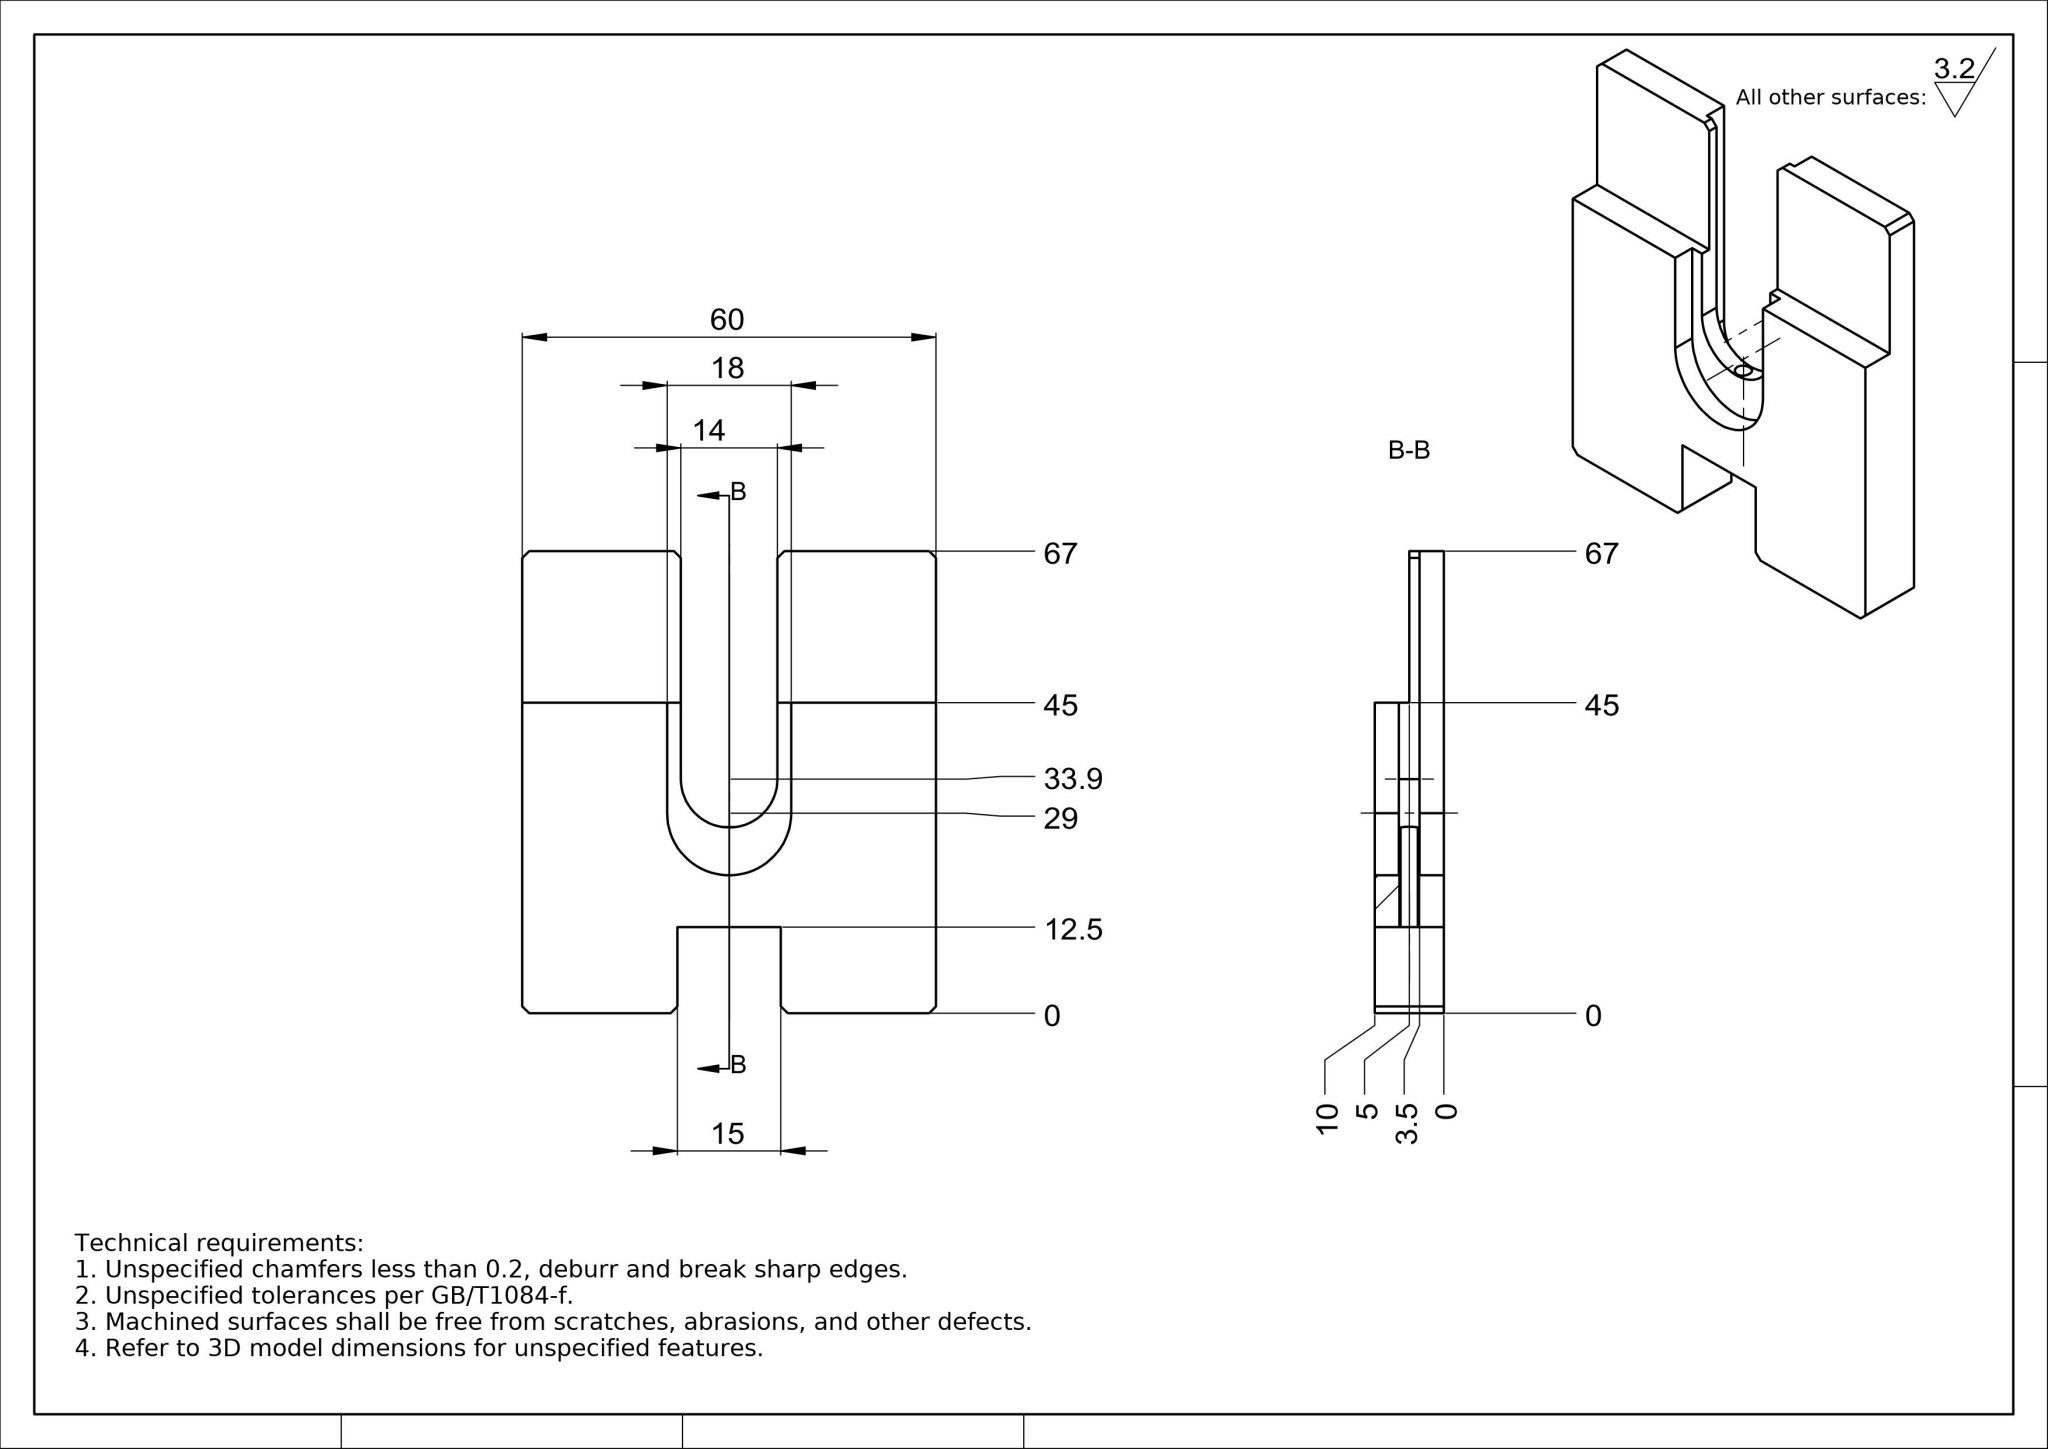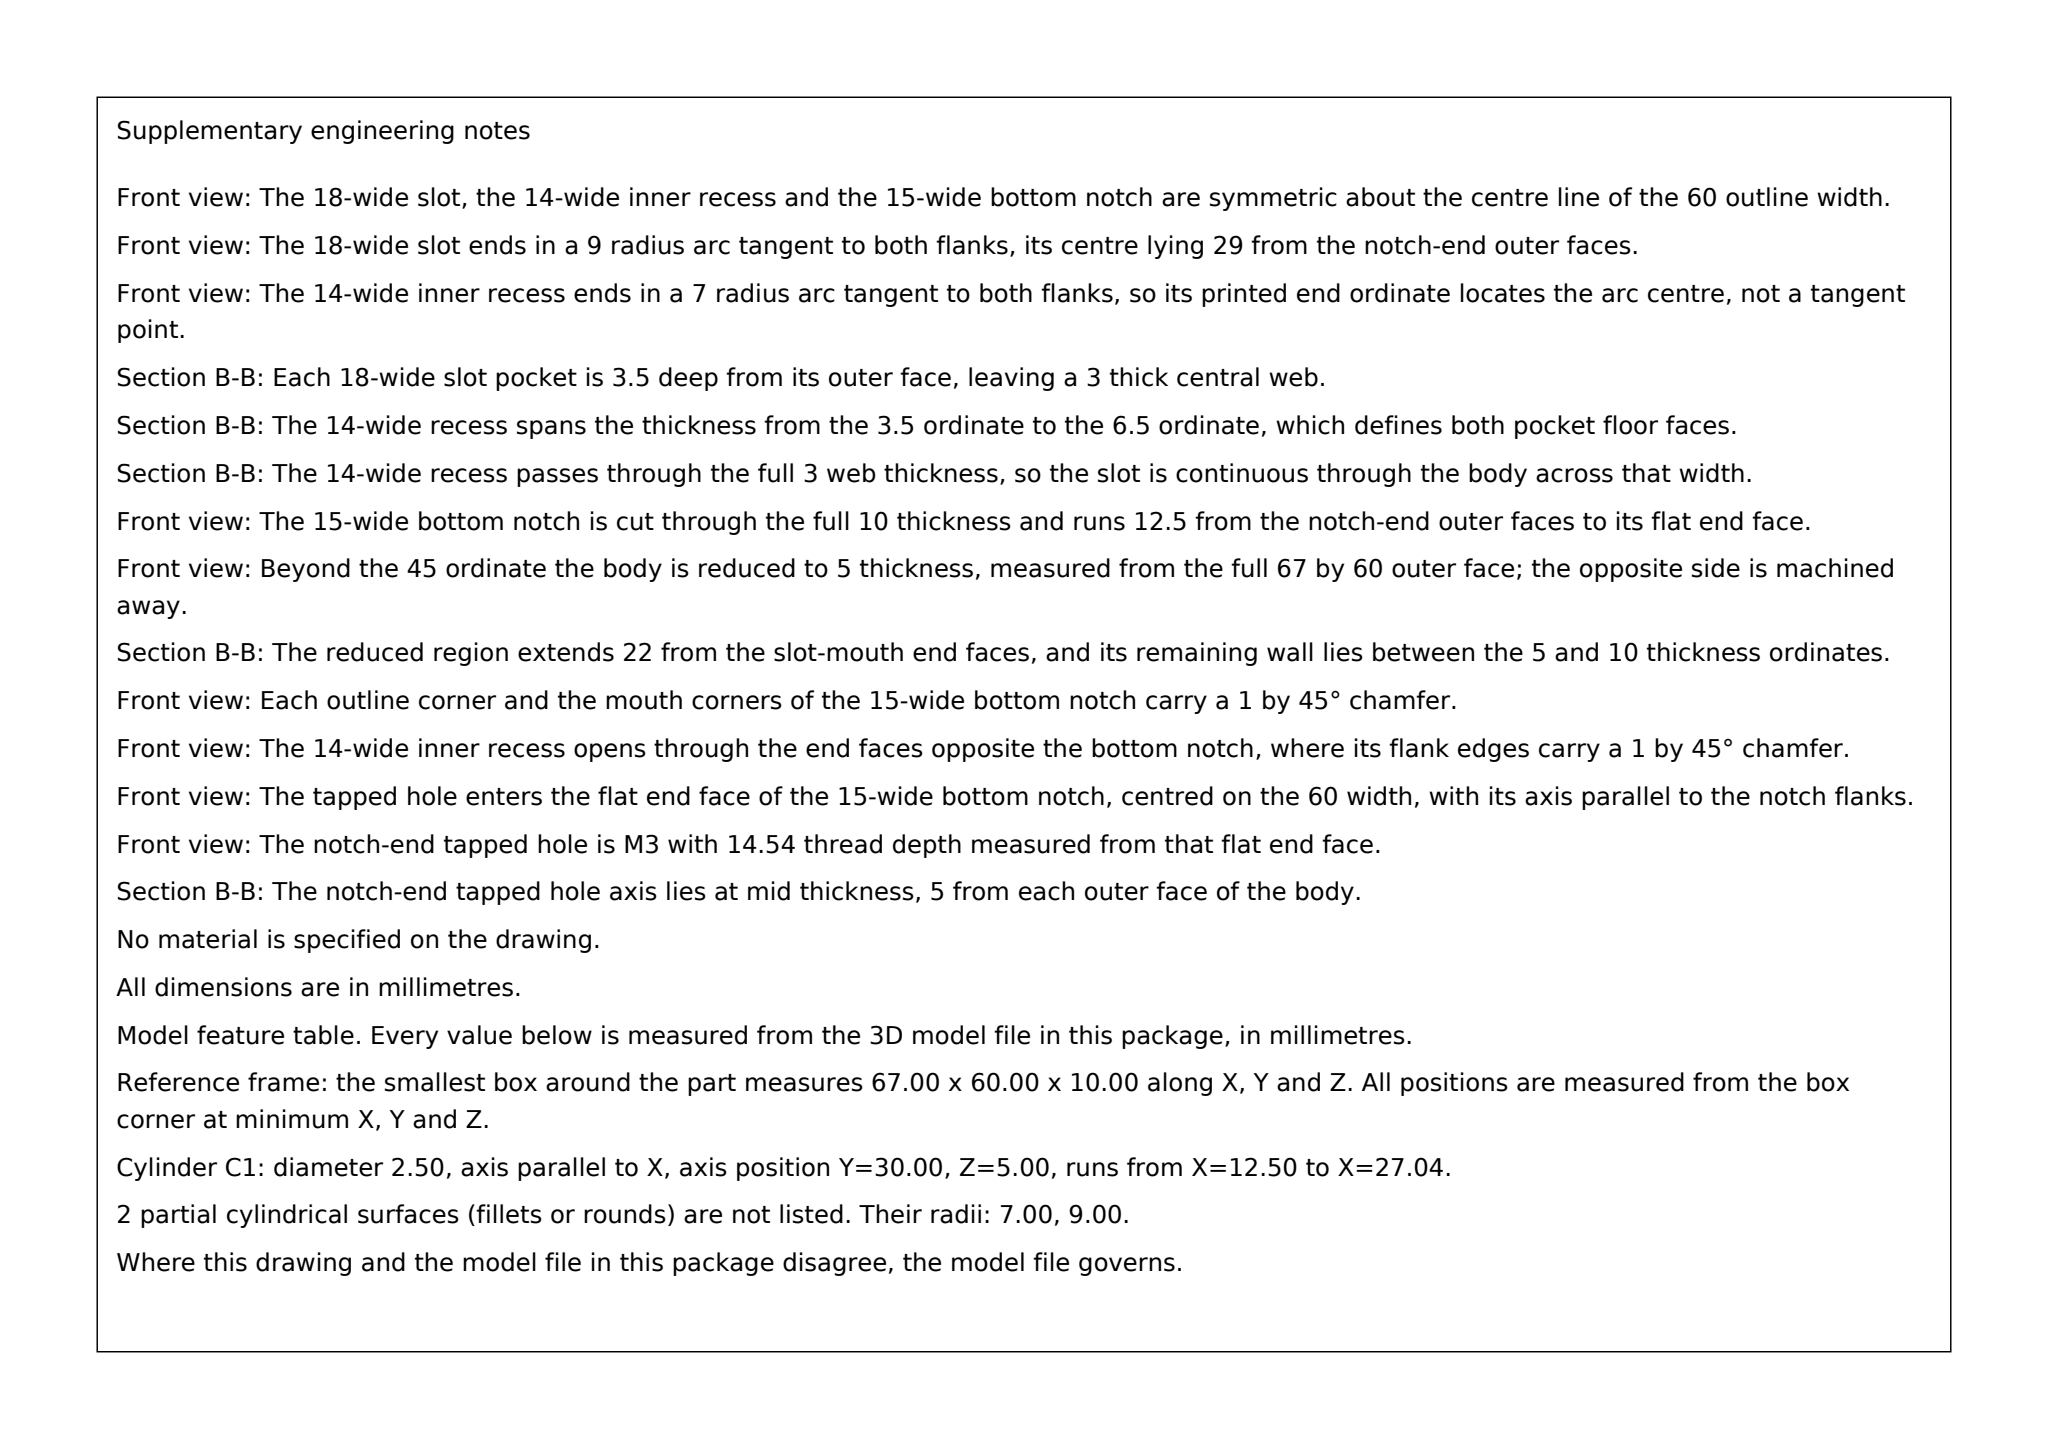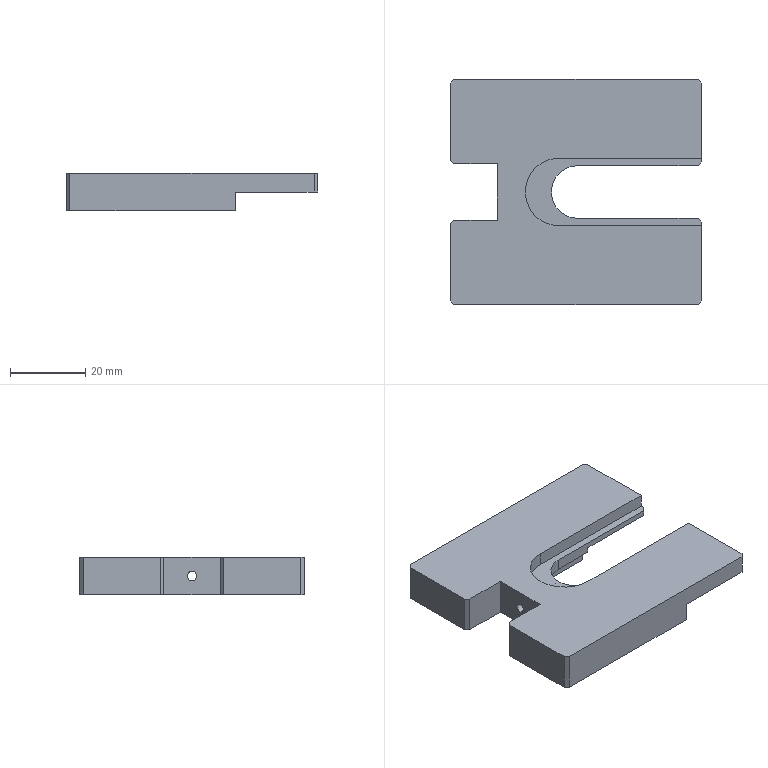Part | SolidWorks | mm | 1 solid | 37 faces | box 67 x 60 x 10 mm | volume 26177 mm3 | plane 31 | cylinder 6 | commonest cylinder face diameters 18 x3 2.5 x2 14 x1
Drawing notes:
Ø2.5 HOLE ON CL AT MID-THK 5: 14.54 LG, FROM 12.5 FACE INTO SLOT | from the solid: cylinders: [2.5,"x",[null,30.0,5.0],14.54,2]; x-planes 12.5; 14-dia slot end at x=33.93 (R7 bottom 26.93); y=30 = CL of 60; z=5 = mid of 10 thk
B-B: 14 U-SLOT POCKET FLOOR AT 6.5; CENTRAL WEB 3 THK (3.5 TO 6.5) | from the solid: z-planes 3.5, 5, 6.5, 10; cylinder [14,"z",[33.93,30.0],len 3.0]; 18-dia pockets 3.5 deep each face
build123d program:
from build123d import *

# Parameters (mm, degrees)
SKETCH1_W           = 67
SKETCH1_H           = 60
BOSS_EXTRUDE1_DEPTH = 5
SKETCH3_W           = 5
SKETCH3_H           = 60
CUT_EXTRUDE1_DEPTH  = 22
CUT_EXTRUDE2_DEPTH  = 3.5
CUT_EXTRUDE3_DEPTH  = 3
SKETCH7_W           = 12.5
SKETCH7_H           = 15
CUT_EXTRUDE4_DEPTH  = 47.068
M3_TAPPED_HOLE1_D   = 2.5
CHAMFER1_SIZE       = 1


with BuildPart() as part:
    # Sketch1 → Boss-Extrude1 (new, symmetric)
    with BuildSketch(Plane.XY):
        Rectangle(SKETCH1_W, SKETCH1_H)
    extrude(amount=BOSS_EXTRUDE1_DEPTH, both=True)

    # Sketch3 → Cut-Extrude1 (cut)
    with BuildSketch(Plane(origin=(33.5, 0, 0), x_dir=(0, 0, -1), z_dir=(1, 0, 0))):
        with Locations((2.5, 0)):
            Rectangle(SKETCH3_W, SKETCH3_H)
    extrude(amount=-CUT_EXTRUDE1_DEPTH, mode=Mode.SUBTRACT)

    # Sketch4 → Cut-Extrude2 (cut)
    with BuildSketch(Plane.XY.offset(5)):
        with BuildLine():
            Line((-4.5, 9), (33.5, 9))
            Line((33.5, 9), (33.5, -9))
            Line((33.5, -9), (-4.5, -9))
            ThreePointArc((-4.5, -9), (-13.5, 0), (-4.5, 9))
        make_face()
    cut_extrude2 = extrude(amount=-CUT_EXTRUDE2_DEPTH, mode=Mode.SUBTRACT)

    # Sketch5 → Cut-Extrude3 (cut)
    with BuildSketch(Plane.XY.offset(1.5)):
        with BuildLine():
            Line((0.43, 7), (43.906, 7))
            Line((43.906, 7), (43.906, -7))
            Line((43.906, -7), (0.43, -7))
            ThreePointArc((0.43, -7), (-6.57, 0), (0.43, 7))
        make_face()
    extrude(amount=-CUT_EXTRUDE3_DEPTH, mode=Mode.SUBTRACT)

    # Mirror1: Cut-Extrude2 across plane
    add(cut_extrude2.mirror(Plane.XY), mode=Mode.SUBTRACT)

    # Sketch7 → Cut-Extrude4 (cut, through all)
    with BuildSketch(Plane.XY.offset(5)):
        with Locations((-27.25, 0)):
            Rectangle(SKETCH7_W, SKETCH7_H)
    extrude(amount=-CUT_EXTRUDE4_DEPTH, mode=Mode.SUBTRACT)

    # M3 Tapped Hole1 (through all)
    with Locations(Plane.ZY.offset(21)):
        with Locations((0, 0)):
            Hole(M3_TAPPED_HOLE1_D / 2)

    # Chamfer1
    chamfer1_edges = [part.edges().sort_by_distance(p)[0] for p in [
        (33.5, 7, 0.75),
        (33.5, -7, 0.75),
        (-33.5, 30, 0),
        (33.5, 30, 2.5),
        (33.5, -30, 2.5),
        (-33.5, -30, 0),
        (-33.5, -7.5, 0),
        (-33.5, 7.5, 0),
    ]]
    chamfer(chamfer1_edges, length=CHAMFER1_SIZE)


solid = part.part